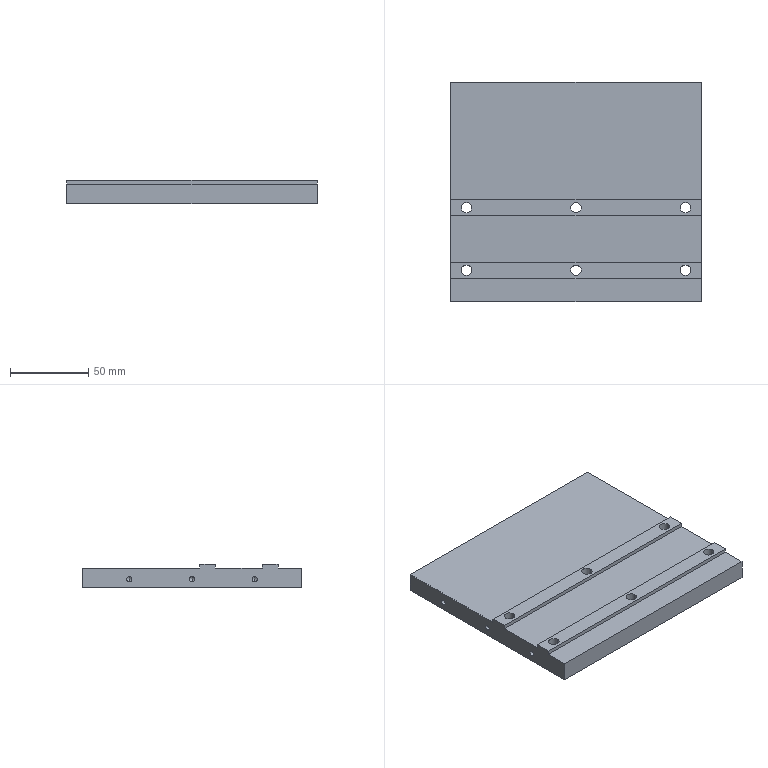Component | SolidWorks | Q1-A12-S21-Q4-03A-6 | 1 solid | 68 faces | box 160 x 140 x 15 mm | volume 281932 mm3 | cylinder 36 | plane 20 | cone 12 | commonest cylinder face diameters 3.3 x12 11 x12 6.6 x12 | material White Plastic Steel POM
build123d program:
from build123d import *

# Parameters (mm, degrees)
SKETCH1_W                                            = 160
SKETCH1_H                                            = 140
BOSS_EXTRUDE1_DEPTH                                  = 15
CYLINDRICAL_COUNTERSUNK_HOLE_FOR_M6_SOCK_D           = 6.6
CYLINDRICAL_COUNTERSUNK_HOLE_FOR_M6_SOCK_CBORE_D     = 11
CYLINDRICAL_COUNTERSUNK_HOLE_FOR_M6_SOCK_CBORE_DEPTH = 6
SKETCH2_W                                            = 2.5
SKETCH2_H                                            = 15
SKETCH2_H_2                                          = 30
SKETCH2_H_3                                          = 75
CUT_EXTRUDE1_DEPTH                                   = 176.285
M4X0_7_TAPPED_HOLE1_D                                = 3.3
M4X0_7_TAPPED_HOLE1_DEPTH                            = 15
M4X0_7_TAPPED_HOLE1_TIP                              = 0.9914
M4X0_7_TAPPED_HOLE2_D                                = 3.3
M4X0_7_TAPPED_HOLE2_DEPTH                            = 15.5
M4X0_7_TAPPED_HOLE2_TIP                              = 0.9914


with BuildPart() as part:
    # Sketch1 → Boss-Extrude1 (new body)
    with BuildSketch(Plane.XY):
        Rectangle(SKETCH1_W, SKETCH1_H)
    extrude(amount=BOSS_EXTRUDE1_DEPTH)

    # Cylindrical Countersunk Hole for M6 Sock (through all)
    with Locations(Plane.XY.offset(15)):
        with Locations((70, -10), (70, -50), (-70, -10), (-70, -50), (0, -10), (0, -50)):
            CounterBoreHole(CYLINDRICAL_COUNTERSUNK_HOLE_FOR_M6_SOCK_D / 2, CYLINDRICAL_COUNTERSUNK_HOLE_FOR_M6_SOCK_CBORE_D / 2, CYLINDRICAL_COUNTERSUNK_HOLE_FOR_M6_SOCK_CBORE_DEPTH)

    # Sketch2 → Cut-Extrude1 (cut, through all)
    with BuildSketch(Plane(origin=(80, 0, 0), x_dir=(0, 0, -1), z_dir=(1, 0, 0))):
        with Locations((-1.25, -62.5)):
            Rectangle(SKETCH2_W, SKETCH2_H)
        with Locations((-1.25, -30)):
            Rectangle(SKETCH2_W, SKETCH2_H_2)
        with Locations((-1.25, 32.5)):
            Rectangle(SKETCH2_W, SKETCH2_H_3)
    extrude(amount=-CUT_EXTRUDE1_DEPTH, mode=Mode.SUBTRACT)

    # M4x0.7 Tapped Hole1
    with Locations(Plane(origin=(80, 0, 0), x_dir=(0, 0, -1), z_dir=(1, 0, 0))):
        with Locations((-9.5, 40), (-9.5, 0), (-9.5, -40)):
            Hole(M4X0_7_TAPPED_HOLE1_D / 2, depth=M4X0_7_TAPPED_HOLE1_DEPTH)
            with Locations((0, 0, -(M4X0_7_TAPPED_HOLE1_DEPTH + M4X0_7_TAPPED_HOLE1_TIP / 2))):  # 118° drill point
                Cone(0, M4X0_7_TAPPED_HOLE1_D / 2, M4X0_7_TAPPED_HOLE1_TIP, mode=Mode.SUBTRACT)

    # M4x0.7 Tapped Hole2
    with Locations(Plane.ZY.offset(80)):
        with Locations((9.5, 40), (9.5, 0), (9.5, -40)):
            Hole(M4X0_7_TAPPED_HOLE2_D / 2, depth=M4X0_7_TAPPED_HOLE2_DEPTH)
            with Locations((0, 0, -(M4X0_7_TAPPED_HOLE2_DEPTH + M4X0_7_TAPPED_HOLE2_TIP / 2))):  # 118° drill point
                Cone(0, M4X0_7_TAPPED_HOLE2_D / 2, M4X0_7_TAPPED_HOLE2_TIP, mode=Mode.SUBTRACT)


solid = part.part

# Placed as in the assembly
solid = solid.moved(Location((1498.5, 30, -147.5), (-180, 0, 180)))